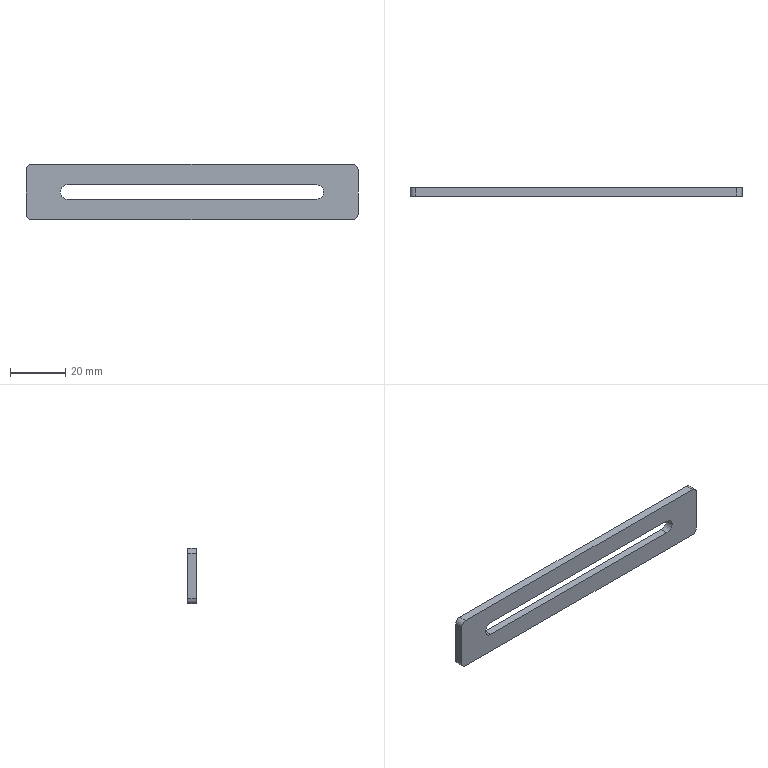Component | SolidWorks | SecondGenerationFour-sidedLabelingTopBatterySidePlate-1 | 1 solid | 15 faces | box 120 x 3 x 20 mm | volume 5722 mm3 | plane 8 | cylinder 7 | commonest cylinder face diameters 4 x4 5.2 x3
build123d program:
from build123d import *

# Parameters (mm, degrees)
SKETCH1_W           = 120
SKETCH1_H           = 20
BOSS_EXTRUDE1_DEPTH = 3
CUT_EXTRUDE1_DEPTH  = 61.902
FILLET1_R           = 2


with BuildPart() as part:
    # Sketch1 → Boss-Extrude1 (new body)
    with BuildSketch(Plane.XY):
        Rectangle(SKETCH1_W, SKETCH1_H)
    extrude(amount=BOSS_EXTRUDE1_DEPTH)

    # Sketch7 → Cut-Extrude1 (cut, through all)
    with BuildSketch(Plane.XY.offset(3)):
        with BuildLine():
            Line((-45, 2.6), (45, 2.6))
            ThreePointArc((45, 2.6), (47.6, 0), (45, -2.6))
            Line((45, -2.6), (-45, -2.6))
            ThreePointArc((-45, -2.6), (-47.6, 0), (-45, 2.6))
        make_face()
    extrude(amount=-CUT_EXTRUDE1_DEPTH, mode=Mode.SUBTRACT)

    # Fillet1
    fillet1_edges = [part.edges().sort_by_distance(p)[0] for p in [
        (60, -10, 1.5),
        (-60, -10, 1.5),
        (-60, 10, 1.5),
        (60, 10, 1.5),
    ]]
    fillet(fillet1_edges, radius=FILLET1_R)


solid = part.part

# Placed as in the assembly
solid = solid.moved(Location((63.358, 46.863, -136.5), (90, 0, 0)))
STEP:
#1=COLOUR_RGB('',0.7922,0.8196,0.9333);
#2=FILL_AREA_STYLE_COLOUR('',#1);
#3=FILL_AREA_STYLE('',(#2));
#4=SURFACE_STYLE_FILL_AREA(#3);
#5=SURFACE_SIDE_STYLE('',(#4));
#6=SURFACE_STYLE_USAGE(.BOTH.,#5);
#7=PRESENTATION_STYLE_ASSIGNMENT((#6));
#8=CARTESIAN_POINT('',(0.6204,1.727,-5.374));
#9=VERTEX_POINT('',#8);
#10=CARTESIAN_POINT('',(0.7227,1.727,-5.272));
#11=VERTEX_POINT('',#10);
#12=CARTESIAN_POINT('',(0.7227,1.727,-5.374));
#13=DIRECTION('',(0.,1.,-0.));
#14=DIRECTION('',(-1.,0.,0.));
#15=AXIS2_PLACEMENT_3D('',#12,#13,#14);
#16=CIRCLE('',#15,0.1024);
#17=EDGE_CURVE('',#9,#11,#16,.T.);
#18=ORIENTED_EDGE('',*,*,#17,.F.);
#19=CARTESIAN_POINT('',(0.6204,1.845,-5.374));
#20=VERTEX_POINT('',#19);
#21=CARTESIAN_POINT('',(0.6204,1.727,-5.374));
#22=DIRECTION('',(0.,1.,-0.));
#23=VECTOR('',#22,39.37);
#24=LINE('',#21,#23);
#25=EDGE_CURVE('',#9,#20,#24,.T.);
#26=ORIENTED_EDGE('',*,*,#25,.T.);
#27=CARTESIAN_POINT('',(0.7227,1.845,-5.272));
#28=VERTEX_POINT('',#27);
#29=CARTESIAN_POINT('',(0.7227,1.845,-5.374));
#30=DIRECTION('',(0.,1.,-0.));
#31=DIRECTION('',(-1.,0.,0.));
#32=AXIS2_PLACEMENT_3D('',#29,#30,#31);
#33=CIRCLE('',#32,0.1024);
#34=EDGE_CURVE('',#20,#28,#33,.T.);
#35=ORIENTED_EDGE('',*,*,#34,.T.);
#36=CARTESIAN_POINT('',(0.7227,1.727,-5.272));
#37=DIRECTION('',(0.,1.,-0.));
#38=VECTOR('',#37,39.37);
#39=LINE('',#36,#38);
#40=EDGE_CURVE('',#11,#28,#39,.T.);
#41=ORIENTED_EDGE('',*,*,#40,.F.);
#42=EDGE_LOOP('',(#18,#26,#35,#41));
#43=FACE_OUTER_BOUND('',#42,.T.);
#44=CARTESIAN_POINT('',(0.7227,1.727,-5.374));
#45=DIRECTION('',(0.,1.,-0.));
#46=DIRECTION('',(-1.,0.,0.));
#47=AXIS2_PLACEMENT_3D('',#44,#45,#46);
#48=CYLINDRICAL_SURFACE('',#47,0.1024);
#49=ADVANCED_FACE('',(#43),#48,.F.);
#50=CARTESIAN_POINT('',(0.1322,1.727,-5.689));
#51=VERTEX_POINT('',#50);
#52=CARTESIAN_POINT('',(0.1322,1.727,-5.059));
#53=VERTEX_POINT('',#52);
#54=CARTESIAN_POINT('',(0.1322,1.727,-5.768));
#55=DIRECTION('',(0.,0.,1.));
#56=VECTOR('',#55,39.37);
#57=LINE('',#54,#56);
#58=EDGE_CURVE('',#51,#53,#57,.T.);
#59=ORIENTED_EDGE('',*,*,#58,.T.);
#60=CARTESIAN_POINT('',(0.1322,1.845,-5.059));
#61=VERTEX_POINT('',#60);
#62=CARTESIAN_POINT('',(0.1322,1.845,-5.059));
#63=DIRECTION('',(0.,1.,-0.));
#64=VECTOR('',#63,39.37);
#65=LINE('',#62,#64);
#66=EDGE_CURVE('',#53,#61,#65,.T.);
#67=ORIENTED_EDGE('',*,*,#66,.T.);
#68=CARTESIAN_POINT('',(0.1322,1.845,-5.689));
#69=VERTEX_POINT('',#68);
#70=CARTESIAN_POINT('',(0.1322,1.845,-5.768));
#71=DIRECTION('',(0.,0.,1.));
#72=VECTOR('',#71,39.37);
#73=LINE('',#70,#72);
#74=EDGE_CURVE('',#69,#61,#73,.T.);
#75=ORIENTED_EDGE('',*,*,#74,.F.);
#76=CARTESIAN_POINT('',(0.1322,1.845,-5.689));
#77=DIRECTION('',(-0.,-1.,0.));
#78=VECTOR('',#77,39.37);
#79=LINE('',#76,#78);
#80=EDGE_CURVE('',#69,#51,#79,.T.);
#81=ORIENTED_EDGE('',*,*,#80,.T.);
#82=EDGE_LOOP('',(#59,#67,#75,#81));
#83=FACE_OUTER_BOUND('',#82,.T.);
#84=CARTESIAN_POINT('',(0.1322,1.845,-5.768));
#85=DIRECTION('',(1.,-0.,-0.));
#86=DIRECTION('',(0.,1.,-0.));
#87=AXIS2_PLACEMENT_3D('',#84,#85,#86);
#88=PLANE('',#87);
#89=ADVANCED_FACE('',(#83),#88,.F.);
#90=CARTESIAN_POINT('',(0.2109,1.845,-4.98));
#91=VERTEX_POINT('',#90);
#92=CARTESIAN_POINT('',(4.778,1.845,-4.98));
#93=VERTEX_POINT('',#92);
#94=CARTESIAN_POINT('',(4.857,1.845,-4.98));
#95=DIRECTION('',(1.,-0.,-0.));
#96=VECTOR('',#95,39.37);
#97=LINE('',#94,#96);
#98=EDGE_CURVE('',#91,#93,#97,.T.);
#99=ORIENTED_EDGE('',*,*,#98,.F.);
#100=CARTESIAN_POINT('',(0.2109,1.727,-4.98));
#101=VERTEX_POINT('',#100);
#102=CARTESIAN_POINT('',(0.2109,1.845,-4.98));
#103=DIRECTION('',(-0.,-1.,0.));
#104=VECTOR('',#103,39.37);
#105=LINE('',#102,#104);
#106=EDGE_CURVE('',#91,#101,#105,.T.);
#107=ORIENTED_EDGE('',*,*,#106,.T.);
#108=CARTESIAN_POINT('',(4.778,1.727,-4.98));
#109=VERTEX_POINT('',#108);
#110=CARTESIAN_POINT('',(4.857,1.727,-4.98));
#111=DIRECTION('',(1.,-0.,-0.));
#112=VECTOR('',#111,39.37);
#113=LINE('',#110,#112);
#114=EDGE_CURVE('',#101,#109,#113,.T.);
#115=ORIENTED_EDGE('',*,*,#114,.T.);
#116=CARTESIAN_POINT('',(4.778,1.845,-4.98));
#117=DIRECTION('',(0.,1.,-0.));
#118=VECTOR('',#117,39.37);
#119=LINE('',#116,#118);
#120=EDGE_CURVE('',#109,#93,#119,.T.);
#121=ORIENTED_EDGE('',*,*,#120,.T.);
#122=EDGE_LOOP('',(#99,#107,#115,#121));
#123=FACE_OUTER_BOUND('',#122,.T.);
#124=CARTESIAN_POINT('',(4.857,1.845,-4.98));
#125=DIRECTION('',(-0.,-0.,-1.));
#126=DIRECTION('',(-0.,-1.,0.));
#127=AXIS2_PLACEMENT_3D('',#124,#125,#126);
#128=PLANE('',#127);
#129=ADVANCED_FACE('',(#123),#128,.F.);
#130=CARTESIAN_POINT('',(4.857,1.727,-5.059));
#131=VERTEX_POINT('',#130);
#132=CARTESIAN_POINT('',(4.857,1.727,-5.689));
#133=VERTEX_POINT('',#132);
#134=CARTESIAN_POINT('',(4.857,1.727,-5.768));
#135=DIRECTION('',(-0.,-0.,-1.));
#136=VECTOR('',#135,39.37);
#137=LINE('',#134,#136);
#138=EDGE_CURVE('',#131,#133,#137,.T.);
#139=ORIENTED_EDGE('',*,*,#138,.T.);
#140=CARTESIAN_POINT('',(4.857,1.845,-5.689));
#141=VERTEX_POINT('',#140);
#142=CARTESIAN_POINT('',(4.857,1.845,-5.689));
#143=DIRECTION('',(0.,1.,-0.));
#144=VECTOR('',#143,39.37);
#145=LINE('',#142,#144);
#146=EDGE_CURVE('',#133,#141,#145,.T.);
#147=ORIENTED_EDGE('',*,*,#146,.T.);
#148=CARTESIAN_POINT('',(4.857,1.845,-5.059));
#149=VERTEX_POINT('',#148);
#150=CARTESIAN_POINT('',(4.857,1.845,-5.768));
#151=DIRECTION('',(-0.,-0.,-1.));
#152=VECTOR('',#151,39.37);
#153=LINE('',#150,#152);
#154=EDGE_CURVE('',#149,#141,#153,.T.);
#155=ORIENTED_EDGE('',*,*,#154,.F.);
#156=CARTESIAN_POINT('',(4.857,1.845,-5.059));
#157=DIRECTION('',(-0.,-1.,0.));
#158=VECTOR('',#157,39.37);
#159=LINE('',#156,#158);
#160=EDGE_CURVE('',#149,#131,#159,.T.);
#161=ORIENTED_EDGE('',*,*,#160,.T.);
#162=EDGE_LOOP('',(#139,#147,#155,#161));
#163=FACE_OUTER_BOUND('',#162,.T.);
#164=CARTESIAN_POINT('',(4.857,1.845,-5.768));
#165=DIRECTION('',(-1.,0.,0.));
#166=DIRECTION('',(-0.,-1.,0.));
#167=AXIS2_PLACEMENT_3D('',#164,#165,#166);
#168=PLANE('',#167);
#169=ADVANCED_FACE('',(#163),#168,.F.);
#170=CARTESIAN_POINT('',(4.778,1.727,-5.768));
#171=VERTEX_POINT('',#170);
#172=CARTESIAN_POINT('',(0.2109,1.727,-5.768));
#173=VERTEX_POINT('',#172);
#174=CARTESIAN_POINT('',(4.857,1.727,-5.768));
#175=DIRECTION('',(-1.,0.,0.));
#176=VECTOR('',#175,39.37);
#177=LINE('',#174,#176);
#178=EDGE_CURVE('',#171,#173,#177,.T.);
#179=ORIENTED_EDGE('',*,*,#178,.T.);
#180=CARTESIAN_POINT('',(0.2109,1.845,-5.768));
#181=VERTEX_POINT('',#180);
#182=CARTESIAN_POINT('',(0.2109,1.845,-5.768));
#183=DIRECTION('',(0.,1.,-0.));
#184=VECTOR('',#183,39.37);
#185=LINE('',#182,#184);
#186=EDGE_CURVE('',#173,#181,#185,.T.);
#187=ORIENTED_EDGE('',*,*,#186,.T.);
#188=CARTESIAN_POINT('',(4.778,1.845,-5.768));
#189=VERTEX_POINT('',#188);
#190=CARTESIAN_POINT('',(4.857,1.845,-5.768));
#191=DIRECTION('',(-1.,0.,0.));
#192=VECTOR('',#191,39.37);
#193=LINE('',#190,#192);
#194=EDGE_CURVE('',#189,#181,#193,.T.);
#195=ORIENTED_EDGE('',*,*,#194,.F.);
#196=CARTESIAN_POINT('',(4.778,1.845,-5.768));
#197=DIRECTION('',(-0.,-1.,0.));
#198=VECTOR('',#197,39.37);
#199=LINE('',#196,#198);
#200=EDGE_CURVE('',#189,#171,#199,.T.);
#201=ORIENTED_EDGE('',*,*,#200,.T.);
#202=EDGE_LOOP('',(#179,#187,#195,#201));
#203=FACE_OUTER_BOUND('',#202,.T.);
#204=CARTESIAN_POINT('',(4.857,1.845,-5.768));
#205=DIRECTION('',(0.,0.,1.));
#206=DIRECTION('',(0.,1.,-0.));
#207=AXIS2_PLACEMENT_3D('',#204,#205,#206);
#208=PLANE('',#207);
#209=ADVANCED_FACE('',(#203),#208,.F.);
#210=CARTESIAN_POINT('',(4.266,1.845,-5.476));
#211=VERTEX_POINT('',#210);
#212=CARTESIAN_POINT('',(0.7227,1.845,-5.476));
#213=VERTEX_POINT('',#212);
#214=CARTESIAN_POINT('',(4.266,1.845,-5.476));
#215=DIRECTION('',(-1.,0.,0.));
#216=VECTOR('',#215,39.37);
#217=LINE('',#214,#216);
#218=EDGE_CURVE('',#211,#213,#217,.T.);
#219=ORIENTED_EDGE('',*,*,#218,.F.);
#220=CARTESIAN_POINT('',(4.266,1.845,-5.272));
#221=VERTEX_POINT('',#220);
#222=CARTESIAN_POINT('',(4.266,1.845,-5.374));
#223=DIRECTION('',(0.,1.,-0.));
#224=DIRECTION('',(-1.,0.,0.));
#225=AXIS2_PLACEMENT_3D('',#222,#223,#224);
#226=CIRCLE('',#225,0.1024);
#227=EDGE_CURVE('',#221,#211,#226,.T.);
#228=ORIENTED_EDGE('',*,*,#227,.F.);
#229=CARTESIAN_POINT('',(4.266,1.845,-5.272));
#230=DIRECTION('',(1.,-0.,-0.));
#231=VECTOR('',#230,39.37);
#232=LINE('',#229,#231);
#233=EDGE_CURVE('',#28,#221,#232,.T.);
#234=ORIENTED_EDGE('',*,*,#233,.F.);
#235=ORIENTED_EDGE('',*,*,#34,.F.);
#236=CARTESIAN_POINT('',(0.7227,1.845,-5.374));
#237=DIRECTION('',(0.,1.,-0.));
#238=DIRECTION('',(-1.,0.,0.));
#239=AXIS2_PLACEMENT_3D('',#236,#237,#238);
#240=CIRCLE('',#239,0.1024);
#241=EDGE_CURVE('',#213,#20,#240,.T.);
#242=ORIENTED_EDGE('',*,*,#241,.F.);
#243=EDGE_LOOP('',(#219,#228,#234,#235,#242));
#244=FACE_BOUND('',#243,.T.);
#245=ORIENTED_EDGE('',*,*,#74,.T.);
#246=CARTESIAN_POINT('',(0.2109,1.845,-5.059));
#247=DIRECTION('',(0.,1.,-0.));
#248=DIRECTION('',(1.,0.,0.));
#249=AXIS2_PLACEMENT_3D('',#246,#247,#248);
#250=CIRCLE('',#249,0.07874);
#251=EDGE_CURVE('',#61,#91,#250,.T.);
#252=ORIENTED_EDGE('',*,*,#251,.T.);
#253=ORIENTED_EDGE('',*,*,#98,.T.);
#254=CARTESIAN_POINT('',(4.778,1.845,-5.059));
#255=DIRECTION('',(0.,1.,-0.));
#256=DIRECTION('',(1.,0.,0.));
#257=AXIS2_PLACEMENT_3D('',#254,#255,#256);
#258=CIRCLE('',#257,0.07874);
#259=EDGE_CURVE('',#93,#149,#258,.T.);
#260=ORIENTED_EDGE('',*,*,#259,.T.);
#261=ORIENTED_EDGE('',*,*,#154,.T.);
#262=CARTESIAN_POINT('',(4.778,1.845,-5.689));
#263=DIRECTION('',(0.,1.,-0.));
#264=DIRECTION('',(1.,0.,0.));
#265=AXIS2_PLACEMENT_3D('',#262,#263,#264);
#266=CIRCLE('',#265,0.07874);
#267=EDGE_CURVE('',#141,#189,#266,.T.);
#268=ORIENTED_EDGE('',*,*,#267,.T.);
#269=ORIENTED_EDGE('',*,*,#194,.T.);
#270=CARTESIAN_POINT('',(0.2109,1.845,-5.689));
#271=DIRECTION('',(0.,1.,-0.));
#272=DIRECTION('',(1.,0.,0.));
#273=AXIS2_PLACEMENT_3D('',#270,#271,#272);
#274=CIRCLE('',#273,0.07874);
#275=EDGE_CURVE('',#181,#69,#274,.T.);
#276=ORIENTED_EDGE('',*,*,#275,.T.);
#277=EDGE_LOOP('',(#245,#252,#253,#260,#261,#268,#269,#276));
#278=FACE_OUTER_BOUND('',#277,.T.);
#279=CARTESIAN_POINT('',(0.1322,1.845,-4.98));
#280=DIRECTION('',(-0.,-1.,0.));
#281=DIRECTION('',(1.,-0.,-0.));
#282=AXIS2_PLACEMENT_3D('',#279,#280,#281);
#283=PLANE('',#282);
#284=ADVANCED_FACE('',(#244,#278),#283,.F.);
#285=CARTESIAN_POINT('',(4.266,1.727,-5.272));
#286=VERTEX_POINT('',#285);
#287=CARTESIAN_POINT('',(4.266,1.727,-5.476));
#288=VERTEX_POINT('',#287);
#289=CARTESIAN_POINT('',(4.266,1.727,-5.374));
#290=DIRECTION('',(0.,1.,-0.));
#291=DIRECTION('',(-1.,0.,0.));
#292=AXIS2_PLACEMENT_3D('',#289,#290,#291);
#293=CIRCLE('',#292,0.1024);
#294=EDGE_CURVE('',#286,#288,#293,.T.);
#295=ORIENTED_EDGE('',*,*,#294,.T.);
#296=CARTESIAN_POINT('',(0.7227,1.727,-5.476));
#297=VERTEX_POINT('',#296);
#298=CARTESIAN_POINT('',(4.266,1.727,-5.476));
#299=DIRECTION('',(-1.,0.,0.));
#300=VECTOR('',#299,39.37);
#301=LINE('',#298,#300);
#302=EDGE_CURVE('',#288,#297,#301,.T.);
#303=ORIENTED_EDGE('',*,*,#302,.T.);
#304=CARTESIAN_POINT('',(0.7227,1.727,-5.374));
#305=DIRECTION('',(0.,1.,-0.));
#306=DIRECTION('',(-1.,0.,0.));
#307=AXIS2_PLACEMENT_3D('',#304,#305,#306);
#308=CIRCLE('',#307,0.1024);
#309=EDGE_CURVE('',#297,#9,#308,.T.);
#310=ORIENTED_EDGE('',*,*,#309,.T.);
#311=ORIENTED_EDGE('',*,*,#17,.T.);
#312=CARTESIAN_POINT('',(4.266,1.727,-5.272));
#313=DIRECTION('',(1.,-0.,-0.));
#314=VECTOR('',#313,39.37);
#315=LINE('',#312,#314);
#316=EDGE_CURVE('',#11,#286,#315,.T.);
#317=ORIENTED_EDGE('',*,*,#316,.T.);
#318=EDGE_LOOP('',(#295,#303,#310,#311,#317));
#319=FACE_BOUND('',#318,.T.);
#320=ORIENTED_EDGE('',*,*,#114,.F.);
#321=CARTESIAN_POINT('',(0.2109,1.727,-5.059));
#322=DIRECTION('',(-0.,-1.,0.));
#323=DIRECTION('',(1.,0.,0.));
#324=AXIS2_PLACEMENT_3D('',#321,#322,#323);
#325=CIRCLE('',#324,0.07874);
#326=EDGE_CURVE('',#101,#53,#325,.T.);
#327=ORIENTED_EDGE('',*,*,#326,.T.);
#328=ORIENTED_EDGE('',*,*,#58,.F.);
#329=CARTESIAN_POINT('',(0.2109,1.727,-5.689));
#330=DIRECTION('',(-0.,-1.,0.));
#331=DIRECTION('',(1.,0.,0.));
#332=AXIS2_PLACEMENT_3D('',#329,#330,#331);
#333=CIRCLE('',#332,0.07874);
#334=EDGE_CURVE('',#51,#173,#333,.T.);
#335=ORIENTED_EDGE('',*,*,#334,.T.);
#336=ORIENTED_EDGE('',*,*,#178,.F.);
#337=CARTESIAN_POINT('',(4.778,1.727,-5.689));
#338=DIRECTION('',(-0.,-1.,0.));
#339=DIRECTION('',(1.,0.,0.));
#340=AXIS2_PLACEMENT_3D('',#337,#338,#339);
#341=CIRCLE('',#340,0.07874);
#342=EDGE_CURVE('',#171,#133,#341,.T.);
#343=ORIENTED_EDGE('',*,*,#342,.T.);
#344=ORIENTED_EDGE('',*,*,#138,.F.);
#345=CARTESIAN_POINT('',(4.778,1.727,-5.059));
#346=DIRECTION('',(-0.,-1.,0.));
#347=DIRECTION('',(1.,0.,0.));
#348=AXIS2_PLACEMENT_3D('',#345,#346,#347);
#349=CIRCLE('',#348,0.07874);
#350=EDGE_CURVE('',#131,#109,#349,.T.);
#351=ORIENTED_EDGE('',*,*,#350,.T.);
#352=EDGE_LOOP('',(#320,#327,#328,#335,#336,#343,#344,#351));
#353=FACE_OUTER_BOUND('',#352,.T.);
#354=CARTESIAN_POINT('',(0.1322,1.727,-4.98));
#355=DIRECTION('',(-0.,-1.,0.));
#356=DIRECTION('',(1.,-0.,-0.));
#357=AXIS2_PLACEMENT_3D('',#354,#355,#356);
#358=PLANE('',#357);
#359=ADVANCED_FACE('',(#319,#353),#358,.T.);
#360=ORIENTED_EDGE('',*,*,#227,.T.);
#361=CARTESIAN_POINT('',(4.266,1.727,-5.476));
#362=DIRECTION('',(0.,1.,-0.));
#363=VECTOR('',#362,39.37);
#364=LINE('',#361,#363);
#365=EDGE_CURVE('',#288,#211,#364,.T.);
#366=ORIENTED_EDGE('',*,*,#365,.F.);
#367=ORIENTED_EDGE('',*,*,#294,.F.);
#368=CARTESIAN_POINT('',(4.266,1.727,-5.272));
#369=DIRECTION('',(0.,1.,-0.));
#370=VECTOR('',#369,39.37);
#371=LINE('',#368,#370);
#372=EDGE_CURVE('',#286,#221,#371,.T.);
#373=ORIENTED_EDGE('',*,*,#372,.T.);
#374=EDGE_LOOP('',(#360,#366,#367,#373));
#375=FACE_OUTER_BOUND('',#374,.T.);
#376=CARTESIAN_POINT('',(4.266,1.727,-5.374));
#377=DIRECTION('',(0.,1.,-0.));
#378=DIRECTION('',(-1.,0.,0.));
#379=AXIS2_PLACEMENT_3D('',#376,#377,#378);
#380=CYLINDRICAL_SURFACE('',#379,0.1024);
#381=ADVANCED_FACE('',(#375),#380,.F.);
#382=ORIENTED_EDGE('',*,*,#233,.T.);
#383=ORIENTED_EDGE('',*,*,#372,.F.);
#384=ORIENTED_EDGE('',*,*,#316,.F.);
#385=ORIENTED_EDGE('',*,*,#40,.T.);
#386=EDGE_LOOP('',(#382,#383,#384,#385));
#387=FACE_OUTER_BOUND('',#386,.T.);
#388=CARTESIAN_POINT('',(4.266,1.727,-5.272));
#389=DIRECTION('',(0.,0.,1.));
#390=DIRECTION('',(0.,1.,-0.));
#391=AXIS2_PLACEMENT_3D('',#388,#389,#390);
#392=PLANE('',#391);
#393=ADVANCED_FACE('',(#387),#392,.F.);
#394=ORIENTED_EDGE('',*,*,#25,.F.);
#395=ORIENTED_EDGE('',*,*,#309,.F.);
#396=CARTESIAN_POINT('',(0.7227,1.727,-5.476));
#397=DIRECTION('',(0.,1.,-0.));
#398=VECTOR('',#397,39.37);
#399=LINE('',#396,#398);
#400=EDGE_CURVE('',#297,#213,#399,.T.);
#401=ORIENTED_EDGE('',*,*,#400,.T.);
#402=ORIENTED_EDGE('',*,*,#241,.T.);
#403=EDGE_LOOP('',(#394,#395,#401,#402));
#404=FACE_OUTER_BOUND('',#403,.T.);
#405=CARTESIAN_POINT('',(0.7227,1.727,-5.374));
#406=DIRECTION('',(0.,1.,-0.));
#407=DIRECTION('',(-1.,0.,0.));
#408=AXIS2_PLACEMENT_3D('',#405,#406,#407);
#409=CYLINDRICAL_SURFACE('',#408,0.1024);
#410=ADVANCED_FACE('',(#404),#409,.F.);
#411=ORIENTED_EDGE('',*,*,#218,.T.);
#412=ORIENTED_EDGE('',*,*,#400,.F.);
#413=ORIENTED_EDGE('',*,*,#302,.F.);
#414=ORIENTED_EDGE('',*,*,#365,.T.);
#415=EDGE_LOOP('',(#411,#412,#413,#414));
#416=FACE_OUTER_BOUND('',#415,.T.);
#417=CARTESIAN_POINT('',(4.266,1.727,-5.476));
#418=DIRECTION('',(-0.,-0.,-1.));
#419=DIRECTION('',(-0.,-1.,0.));
#420=AXIS2_PLACEMENT_3D('',#417,#418,#419);
#421=PLANE('',#420);
#422=ADVANCED_FACE('',(#416),#421,.F.);
#423=ORIENTED_EDGE('',*,*,#251,.F.);
#424=ORIENTED_EDGE('',*,*,#66,.F.);
#425=ORIENTED_EDGE('',*,*,#326,.F.);
#426=ORIENTED_EDGE('',*,*,#106,.F.);
#427=EDGE_LOOP('',(#423,#424,#425,#426));
#428=FACE_OUTER_BOUND('',#427,.T.);
#429=CARTESIAN_POINT('',(0.2109,1.845,-5.059));
#430=DIRECTION('',(-0.,-1.,0.));
#431=DIRECTION('',(1.,0.,0.));
#432=AXIS2_PLACEMENT_3D('',#429,#430,#431);
#433=CYLINDRICAL_SURFACE('',#432,0.07874);
#434=ADVANCED_FACE('',(#428),#433,.T.);
#435=ORIENTED_EDGE('',*,*,#275,.F.);
#436=ORIENTED_EDGE('',*,*,#186,.F.);
#437=ORIENTED_EDGE('',*,*,#334,.F.);
#438=ORIENTED_EDGE('',*,*,#80,.F.);
#439=EDGE_LOOP('',(#435,#436,#437,#438));
#440=FACE_OUTER_BOUND('',#439,.T.);
#441=CARTESIAN_POINT('',(0.2109,1.845,-5.689));
#442=DIRECTION('',(-0.,-1.,0.));
#443=DIRECTION('',(1.,0.,0.));
#444=AXIS2_PLACEMENT_3D('',#441,#442,#443);
#445=CYLINDRICAL_SURFACE('',#444,0.07874);
#446=ADVANCED_FACE('',(#440),#445,.T.);
#447=ORIENTED_EDGE('',*,*,#267,.F.);
#448=ORIENTED_EDGE('',*,*,#146,.F.);
#449=ORIENTED_EDGE('',*,*,#342,.F.);
#450=ORIENTED_EDGE('',*,*,#200,.F.);
#451=EDGE_LOOP('',(#447,#448,#449,#450));
#452=FACE_OUTER_BOUND('',#451,.T.);
#453=CARTESIAN_POINT('',(4.778,1.845,-5.689));
#454=DIRECTION('',(-0.,-1.,0.));
#455=DIRECTION('',(1.,0.,0.));
#456=AXIS2_PLACEMENT_3D('',#453,#454,#455);
#457=CYLINDRICAL_SURFACE('',#456,0.07874);
#458=ADVANCED_FACE('',(#452),#457,.T.);
#459=ORIENTED_EDGE('',*,*,#259,.F.);
#460=ORIENTED_EDGE('',*,*,#120,.F.);
#461=ORIENTED_EDGE('',*,*,#350,.F.);
#462=ORIENTED_EDGE('',*,*,#160,.F.);
#463=EDGE_LOOP('',(#459,#460,#461,#462));
#464=FACE_OUTER_BOUND('',#463,.T.);
#465=CARTESIAN_POINT('',(4.778,1.845,-5.059));
#466=DIRECTION('',(-0.,-1.,0.));
#467=DIRECTION('',(1.,0.,0.));
#468=AXIS2_PLACEMENT_3D('',#465,#466,#467);
#469=CYLINDRICAL_SURFACE('',#468,0.07874);
#470=ADVANCED_FACE('',(#464),#469,.T.);
#471=CLOSED_SHELL('',(#49,#89,#129,#169,#209,#284,#359,#381,#393,#410,#422,#434,#446,#458,#470));
#472=MANIFOLD_SOLID_BREP('',#471);
#473=STYLED_ITEM('',(#7),#472);
#474=PRESENTATION_LAYER_ASSIGNMENT('','',(#473));
#475=(LENGTH_UNIT()NAMED_UNIT(*)SI_UNIT($,.METRE.));
#476=LENGTH_MEASURE_WITH_UNIT(LENGTH_MEASURE(0.0254),#475);
#477=DIMENSIONAL_EXPONENTS(1.,0.,0.,0.,0.,0.,0.);
#478=(CONVERSION_BASED_UNIT('',#476)LENGTH_UNIT()NAMED_UNIT(#477));
#479=UNCERTAINTY_MEASURE_WITH_UNIT(LENGTH_MEASURE(0.00001),#478,'','');
#480=(NAMED_UNIT(*)PLANE_ANGLE_UNIT()SI_UNIT($,.RADIAN.));
#481=(NAMED_UNIT(*)SI_UNIT($,.STERADIAN.)SOLID_ANGLE_UNIT());
#482=(GEOMETRIC_REPRESENTATION_CONTEXT(3)GLOBAL_UNCERTAINTY_ASSIGNED_CONTEXT((#479))GLOBAL_UNIT_ASSIGNED_CONTEXT((#478,#480,#481))REPRESENTATION_CONTEXT('',''));
#483=MECHANICAL_DESIGN_GEOMETRIC_PRESENTATION_REPRESENTATION('',(#473),#482);
#484=CARTESIAN_POINT('',(0.,0.,0.));
#485=DIRECTION('',(0.,0.,1.));
#486=DIRECTION('',(1.,0.,0.));
#487=AXIS2_PLACEMENT_3D('',#484,#485,#486);
#488=(LENGTH_UNIT()NAMED_UNIT(*)SI_UNIT($,.METRE.));
#489=LENGTH_MEASURE_WITH_UNIT(LENGTH_MEASURE(0.0254),#488);
#490=DIMENSIONAL_EXPONENTS(1.,0.,0.,0.,0.,0.,0.);
#491=(CONVERSION_BASED_UNIT('',#489)LENGTH_UNIT()NAMED_UNIT(#490));
#492=UNCERTAINTY_MEASURE_WITH_UNIT(LENGTH_MEASURE(0.00001),#491,'','');
#493=(NAMED_UNIT(*)PLANE_ANGLE_UNIT()SI_UNIT($,.RADIAN.));
#494=(NAMED_UNIT(*)SI_UNIT($,.STERADIAN.)SOLID_ANGLE_UNIT());
#495=(GEOMETRIC_REPRESENTATION_CONTEXT(3)GLOBAL_UNCERTAINTY_ASSIGNED_CONTEXT((#492))GLOBAL_UNIT_ASSIGNED_CONTEXT((#491,#493,#494))REPRESENTATION_CONTEXT('',''));
#496=ADVANCED_BREP_SHAPE_REPRESENTATION('',(#472,#487),#495);